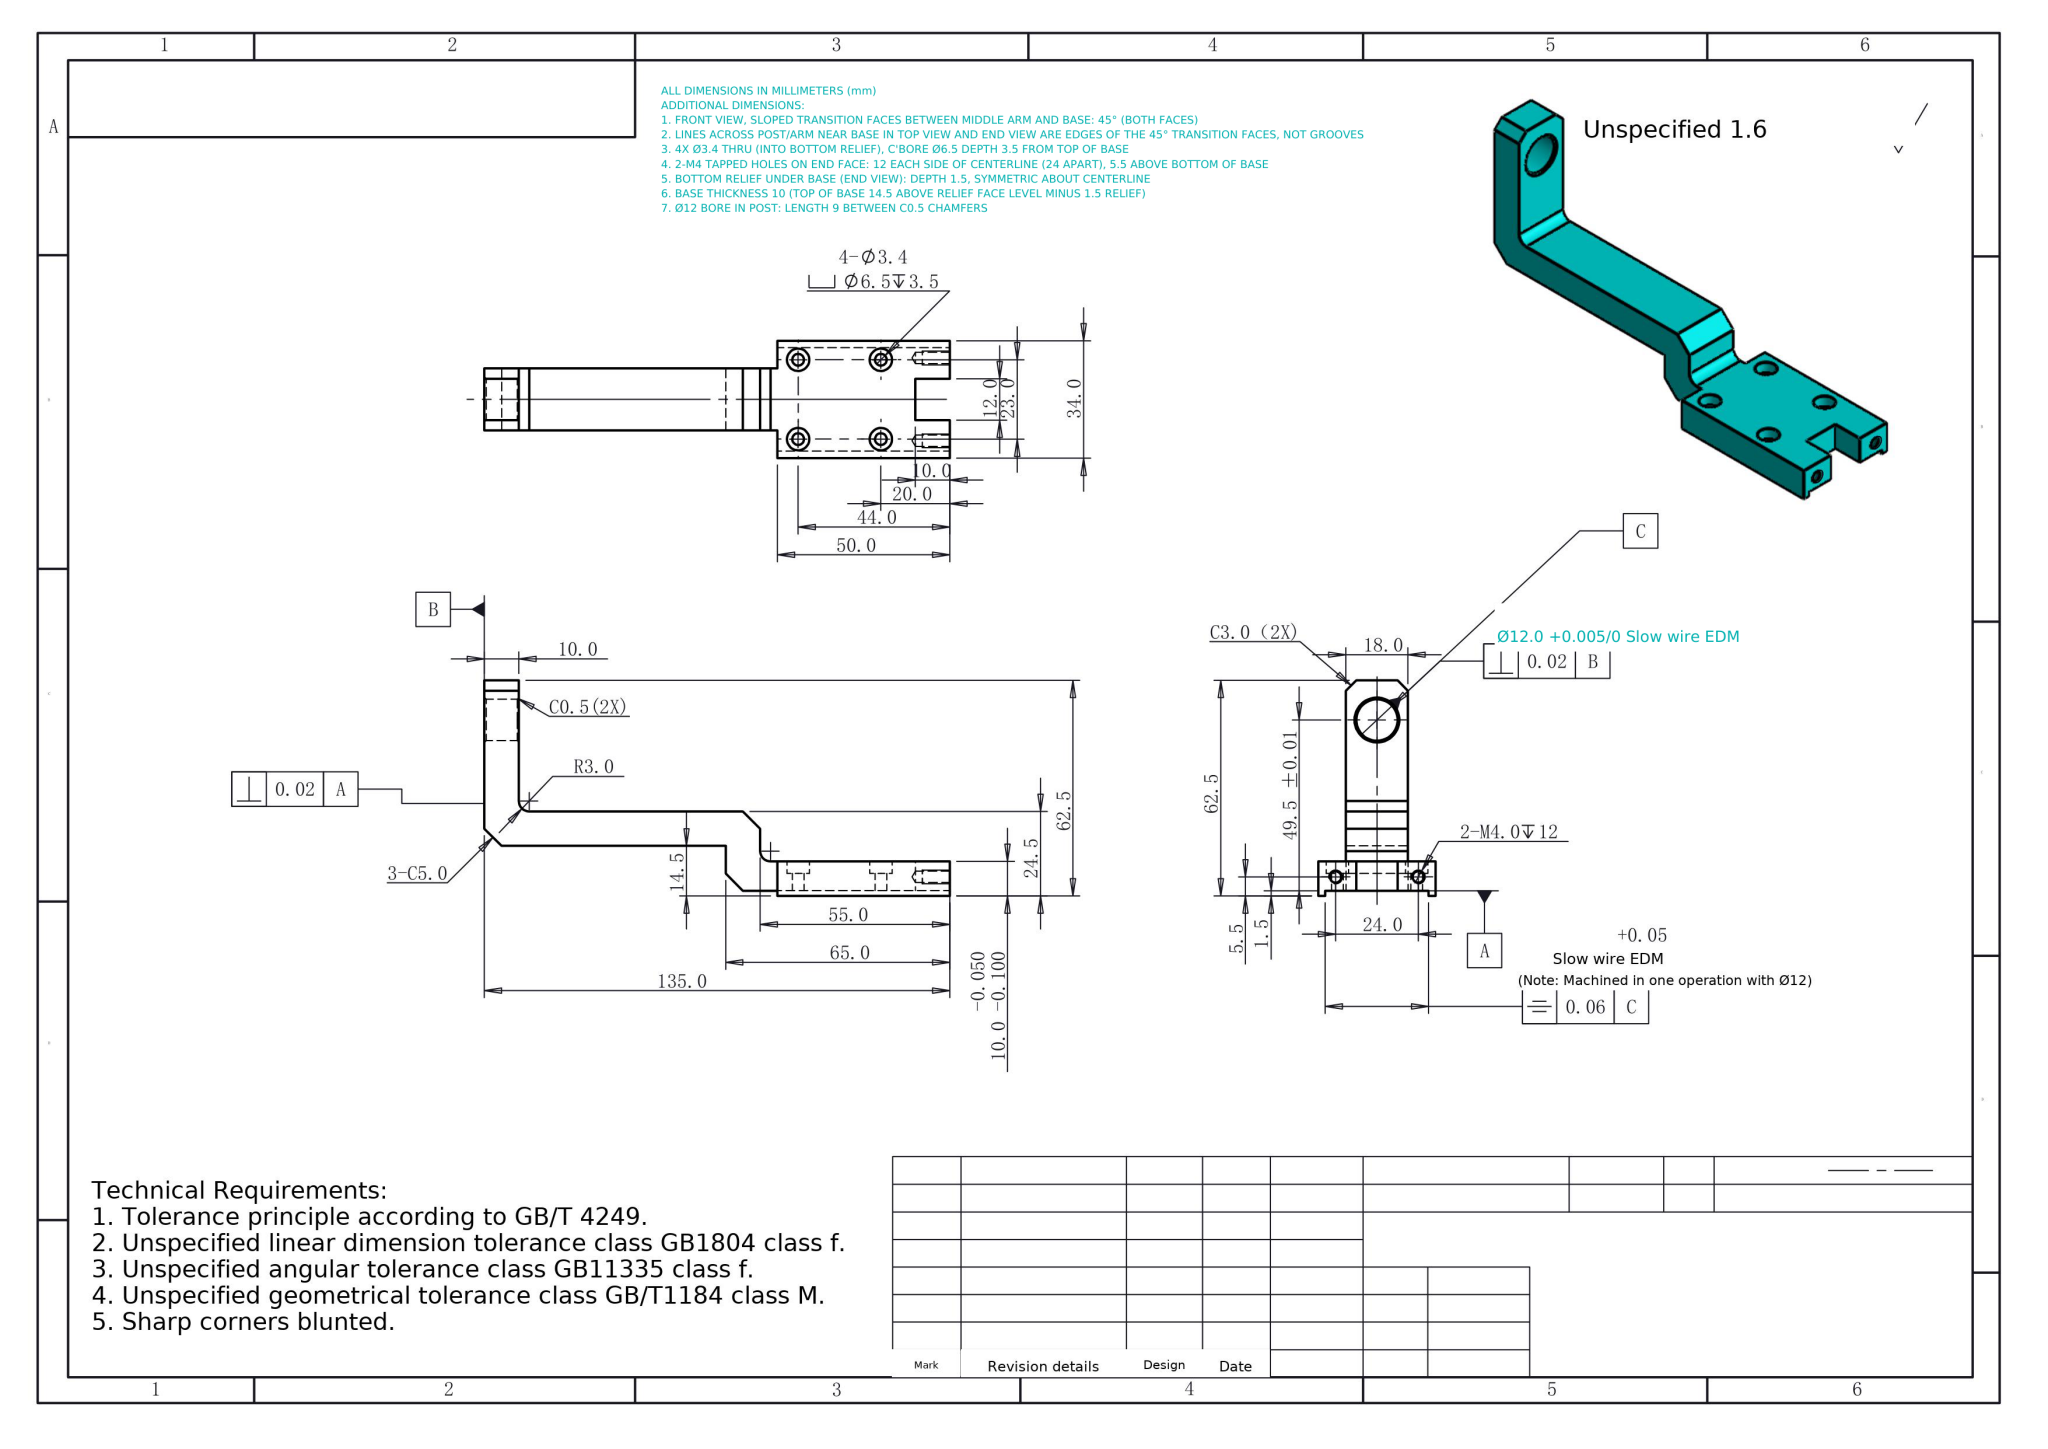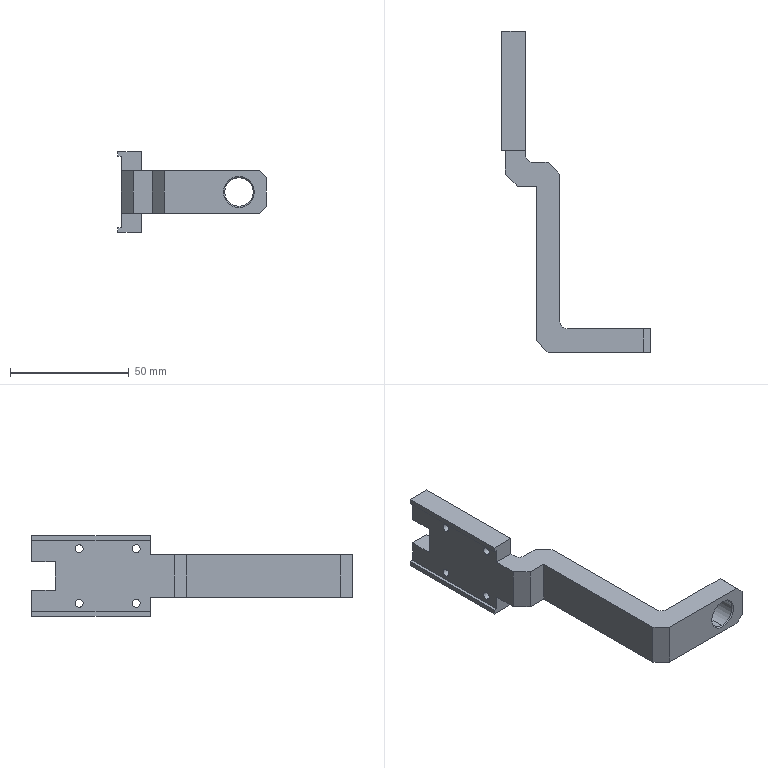Part | NX | mm | 1 solid | 65 faces | box 62.5 x 135 x 34 mm | volume 35416 mm3 | plane 33 | cylinder 24 | cone 8 | commonest cylinder face diameters 6.5 x8 3.4 x8 3.3 x4 12 x2 6 x2